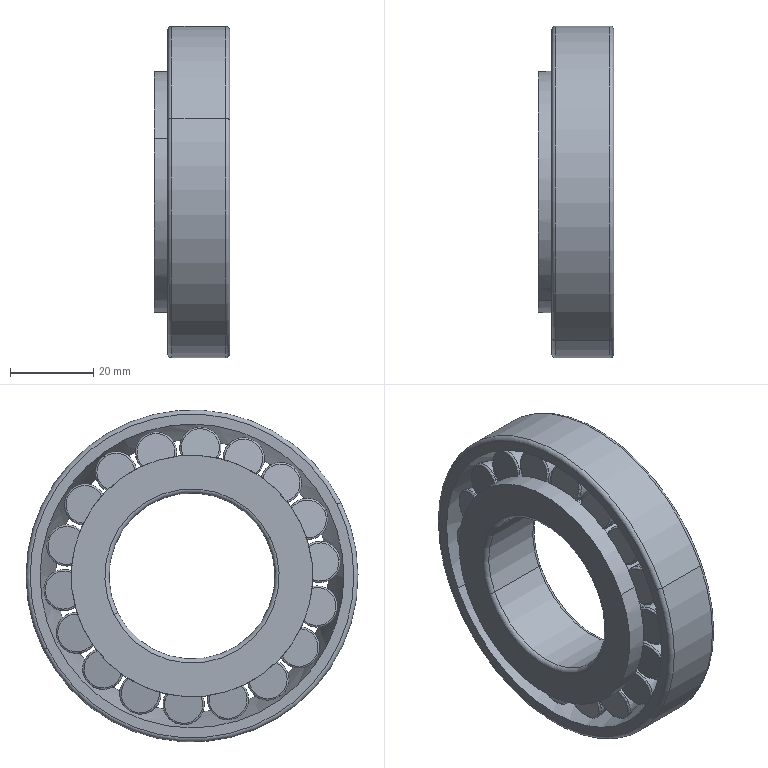Component | SolidWorks | tapered roller bearings gb 40x80x18.25-1 | 1 solid | 172 faces | volume 47697 mm3 | torus 80 | cone 44 | plane 40 | cylinder 8 | commonest cylinder face diameters 80 x2 53.701 x2 58.177 x2 40 x2